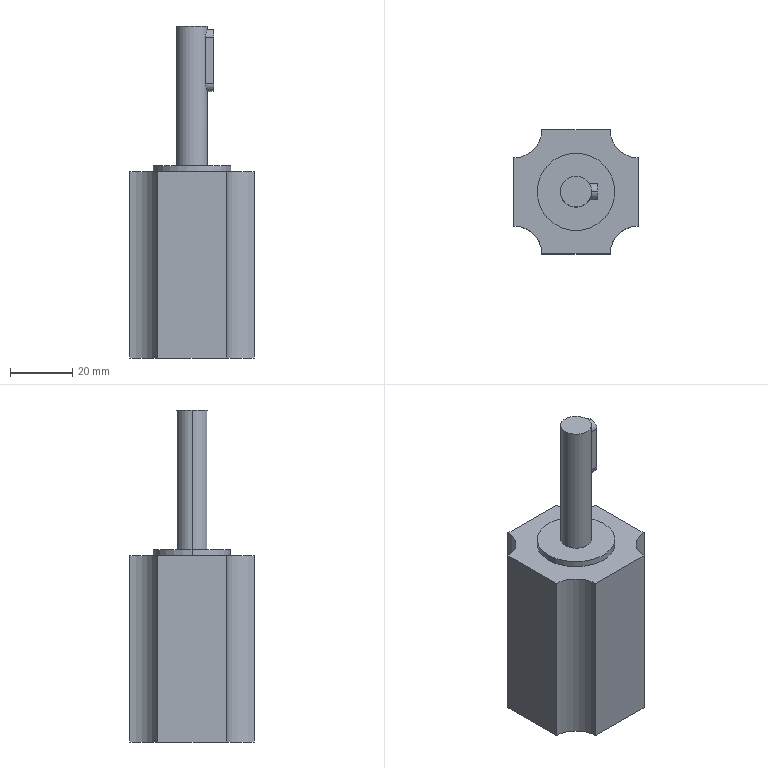Component | SolidWorks | FormingWheelMotor-1 | 1 solid | 22 faces | box 40 x 40 x 107 mm | volume 85457 mm3 | cylinder 11 | plane 11 | commonest cylinder face diameters 18 x4 5 x3 25 x2 10 x2
build123d program:
from build123d import *

# Parameters (mm, degrees)
SKETCH1_R           = 5
BOSS_EXTRUDE1_DEPTH = 45
SKETCH4_R           = 12.5
BOSS_EXTRUDE2_DEPTH = 2
SKETCH5_W           = 40
SKETCH5_H           = 40
BOSS_EXTRUDE3_DEPTH = 60
SKETCH6_R           = 9
CUT_EXTRUDE2_DEPTH  = 111.675
BOSS_EXTRUDE4_DEPTH = 7


with BuildPart() as part:
    # Sketch1 → Boss-Extrude1 (new body)
    with BuildSketch(Plane(origin=(0, 0, 0), x_dir=(0, 0, -1), z_dir=(1, 0, 0))):
        with Locations(Location((0, 0, 0), (0, 0, 180))):
            Circle(SKETCH1_R)
    extrude(amount=BOSS_EXTRUDE1_DEPTH)

    # Sketch4 → Boss-Extrude2 (add)
    with BuildSketch(Plane(origin=(45, 0, 0), x_dir=(0, 0, -1), z_dir=(1, 0, 0))):
        Circle(SKETCH4_R)
    extrude(amount=BOSS_EXTRUDE2_DEPTH)

    # Sketch5 → Boss-Extrude3 (add)
    with BuildSketch(Plane(origin=(47, 0, 0), x_dir=(0, 0, -1), z_dir=(1, 0, 0))):
        Rectangle(SKETCH5_W, SKETCH5_H)
    extrude(amount=BOSS_EXTRUDE3_DEPTH)

    # Sketch6 → Cut-Extrude2 (cut, through all)
    with BuildSketch(Plane(origin=(107, 0, 0), x_dir=(0, 0, -1), z_dir=(1, 0, 0))):
        with Locations((-20, 20)):
            Circle(SKETCH6_R)
        with Locations((20, 20)):
            Circle(SKETCH6_R)
        with Locations((20, -20)):
            Circle(SKETCH6_R)
        with Locations((-20, -20)):
            Circle(SKETCH6_R)
    extrude(amount=-CUT_EXTRUDE2_DEPTH, mode=Mode.SUBTRACT)

    # Sketch3 → Boss-Extrude4 (add)
    with BuildSketch(Plane.XY):
        with BuildLine():
            Line((3.623, 2.5), (18.623, 2.5))
            ThreePointArc((18.623, 2.5), (21.123, 0), (18.623, -2.5))
            Line((18.623, -2.5), (3.623, -2.5))
            ThreePointArc((3.623, -2.5), (1.123, 0), (3.623, 2.5))
        make_face()
    extrude(amount=BOSS_EXTRUDE4_DEPTH)


solid = part.part

# Placed as in the assembly
solid = solid.moved(Location((246.241, -267.715, 1455.724), (0, 90, 0)))
STEP:
#1=CARTESIAN_POINT('',(9.97,-10.54,57.268));
#2=VERTEX_POINT('',#1);
#3=CARTESIAN_POINT('',(9.97,-10.638,57.169));
#4=VERTEX_POINT('',#3);
#5=CARTESIAN_POINT('',(9.97,-10.54,57.169));
#6=DIRECTION('',(1.,0.,-0.));
#7=DIRECTION('',(0.,0.,-1.));
#8=AXIS2_PLACEMENT_3D('',#5,#6,#7);
#9=CIRCLE('',#8,0.09843);
#10=EDGE_CURVE('',#2,#4,#9,.T.);
#11=ORIENTED_EDGE('',*,*,#10,.F.);
#12=CARTESIAN_POINT('',(9.891,-10.54,57.268));
#13=VERTEX_POINT('',#12);
#14=CARTESIAN_POINT('',(9.97,-10.54,57.268));
#15=DIRECTION('',(-1.,-0.,0.));
#16=VECTOR('',#15,39.37);
#17=LINE('',#14,#16);
#18=EDGE_CURVE('',#2,#13,#17,.T.);
#19=ORIENTED_EDGE('',*,*,#18,.T.);
#20=CARTESIAN_POINT('',(9.865,-10.638,57.169));
#21=VERTEX_POINT('',#20);
#22=CARTESIAN_POINT('',(9.891,-10.54,57.268));
#23=CARTESIAN_POINT('',(9.891,-10.546,57.268));
#24=CARTESIAN_POINT('',(9.891,-10.553,57.267));
#25=CARTESIAN_POINT('',(9.89,-10.566,57.265));
#26=CARTESIAN_POINT('',(9.889,-10.572,57.263));
#27=CARTESIAN_POINT('',(9.886,-10.584,57.258));
#28=CARTESIAN_POINT('',(9.885,-10.59,57.255));
#29=CARTESIAN_POINT('',(9.882,-10.6,57.247));
#30=CARTESIAN_POINT('',(9.88,-10.605,57.243));
#31=CARTESIAN_POINT('',(9.877,-10.614,57.234));
#32=CARTESIAN_POINT('',(9.875,-10.618,57.229));
#33=CARTESIAN_POINT('',(9.872,-10.625,57.219));
#34=CARTESIAN_POINT('',(9.87,-10.628,57.213));
#35=CARTESIAN_POINT('',(9.868,-10.633,57.201));
#36=CARTESIAN_POINT('',(9.867,-10.635,57.195));
#37=CARTESIAN_POINT('',(9.865,-10.638,57.182));
#38=CARTESIAN_POINT('',(9.865,-10.638,57.176));
#39=CARTESIAN_POINT('',(9.865,-10.638,57.169));
#40=B_SPLINE_CURVE_WITH_KNOTS('',3,(#22,#23,#24,#25,#26,#27,#28,#29,#30,#31,#32,#33,#34,#35,#36,#37,#38,#39),.UNSPECIFIED.,.F.,.F.,(4,2,2,2,2,2,2,2,4),(0.007952,0.008449,0.008945,0.009442,0.009938,0.01043,0.01093,0.01143,0.01192),.UNSPECIFIED.);
#41=EDGE_CURVE('',#13,#21,#40,.T.);
#42=ORIENTED_EDGE('',*,*,#41,.T.);
#43=CARTESIAN_POINT('',(9.97,-10.638,57.169));
#44=DIRECTION('',(-1.,-0.,0.));
#45=VECTOR('',#44,39.37);
#46=LINE('',#43,#45);
#47=EDGE_CURVE('',#4,#21,#46,.T.);
#48=ORIENTED_EDGE('',*,*,#47,.F.);
#49=EDGE_LOOP('',(#11,#19,#42,#48));
#50=FACE_OUTER_BOUND('',#49,.T.);
#51=CARTESIAN_POINT('',(9.97,-10.54,57.169));
#52=DIRECTION('',(-1.,-0.,0.));
#53=DIRECTION('',(0.,0.,1.));
#54=AXIS2_PLACEMENT_3D('',#51,#52,#53);
#55=CYLINDRICAL_SURFACE('',#54,0.09843);
#56=ADVANCED_FACE('',(#50),#55,.T.);
#57=CARTESIAN_POINT('',(9.202,-10.54,55.462));
#58=VERTEX_POINT('',#57);
#59=CARTESIAN_POINT('',(10.187,-10.54,55.462));
#60=VERTEX_POINT('',#59);
#61=CARTESIAN_POINT('',(9.695,-10.54,55.462));
#62=DIRECTION('',(-0.,0.,-1.));
#63=DIRECTION('',(-1.,0.,0.));
#64=AXIS2_PLACEMENT_3D('',#61,#62,#63);
#65=CIRCLE('',#64,0.4921);
#66=EDGE_CURVE('',#58,#60,#65,.T.);
#67=ORIENTED_EDGE('',*,*,#66,.F.);
#68=CARTESIAN_POINT('',(9.202,-10.54,55.54));
#69=VERTEX_POINT('',#68);
#70=CARTESIAN_POINT('',(9.202,-10.54,55.462));
#71=DIRECTION('',(0.,-0.,1.));
#72=VECTOR('',#71,39.37);
#73=LINE('',#70,#72);
#74=EDGE_CURVE('',#58,#69,#73,.T.);
#75=ORIENTED_EDGE('',*,*,#74,.T.);
#76=CARTESIAN_POINT('',(10.187,-10.54,55.54));
#77=VERTEX_POINT('',#76);
#78=CARTESIAN_POINT('',(9.695,-10.54,55.54));
#79=DIRECTION('',(-0.,0.,-1.));
#80=DIRECTION('',(-1.,0.,0.));
#81=AXIS2_PLACEMENT_3D('',#78,#79,#80);
#82=CIRCLE('',#81,0.4921);
#83=EDGE_CURVE('',#69,#77,#82,.T.);
#84=ORIENTED_EDGE('',*,*,#83,.T.);
#85=CARTESIAN_POINT('',(10.187,-10.54,55.462));
#86=DIRECTION('',(0.,-0.,1.));
#87=VECTOR('',#86,39.37);
#88=LINE('',#85,#87);
#89=EDGE_CURVE('',#60,#77,#88,.T.);
#90=ORIENTED_EDGE('',*,*,#89,.F.);
#91=EDGE_LOOP('',(#67,#75,#84,#90));
#92=FACE_OUTER_BOUND('',#91,.T.);
#93=CARTESIAN_POINT('',(9.695,-10.54,55.462));
#94=DIRECTION('',(0.,-0.,1.));
#95=DIRECTION('',(1.,0.,0.));
#96=AXIS2_PLACEMENT_3D('',#93,#94,#95);
#97=CYLINDRICAL_SURFACE('',#96,0.4921);
#98=ADVANCED_FACE('',(#92),#97,.T.);
#99=CARTESIAN_POINT('',(9.498,-10.54,55.54));
#100=VERTEX_POINT('',#99);
#101=CARTESIAN_POINT('',(9.891,-10.54,55.54));
#102=VERTEX_POINT('',#101);
#103=CARTESIAN_POINT('',(9.695,-10.54,55.54));
#104=DIRECTION('',(-0.,0.,-1.));
#105=DIRECTION('',(-1.,0.,0.));
#106=AXIS2_PLACEMENT_3D('',#103,#104,#105);
#107=CIRCLE('',#106,0.1969);
#108=EDGE_CURVE('',#100,#102,#107,.T.);
#109=ORIENTED_EDGE('',*,*,#108,.F.);
#110=CARTESIAN_POINT('',(9.498,-10.54,57.312));
#111=VERTEX_POINT('',#110);
#112=CARTESIAN_POINT('',(9.498,-10.54,55.54));
#113=DIRECTION('',(0.,-0.,1.));
#114=VECTOR('',#113,39.37);
#115=LINE('',#112,#114);
#116=EDGE_CURVE('',#100,#111,#115,.T.);
#117=ORIENTED_EDGE('',*,*,#116,.T.);
#118=CARTESIAN_POINT('',(9.891,-10.54,57.312));
#119=VERTEX_POINT('',#118);
#120=CARTESIAN_POINT('',(9.695,-10.54,57.312));
#121=DIRECTION('',(-0.,0.,-1.));
#122=DIRECTION('',(-1.,0.,0.));
#123=AXIS2_PLACEMENT_3D('',#120,#121,#122);
#124=CIRCLE('',#123,0.1969);
#125=EDGE_CURVE('',#111,#119,#124,.T.);
#126=ORIENTED_EDGE('',*,*,#125,.T.);
#127=CARTESIAN_POINT('',(9.891,-10.54,55.54));
#128=DIRECTION('',(0.,-0.,1.));
#129=VECTOR('',#128,39.37);
#130=LINE('',#127,#129);
#131=EDGE_CURVE('',#13,#119,#130,.T.);
#132=ORIENTED_EDGE('',*,*,#131,.F.);
#133=CARTESIAN_POINT('',(9.865,-10.442,57.169));
#134=VERTEX_POINT('',#133);
#135=CARTESIAN_POINT('',(9.865,-10.442,57.169));
#136=CARTESIAN_POINT('',(9.865,-10.442,57.176));
#137=CARTESIAN_POINT('',(9.865,-10.442,57.183));
#138=CARTESIAN_POINT('',(9.867,-10.445,57.195));
#139=CARTESIAN_POINT('',(9.868,-10.447,57.202));
#140=CARTESIAN_POINT('',(9.871,-10.452,57.213));
#141=CARTESIAN_POINT('',(9.872,-10.455,57.219));
#142=CARTESIAN_POINT('',(9.875,-10.462,57.23));
#143=CARTESIAN_POINT('',(9.877,-10.466,57.235));
#144=CARTESIAN_POINT('',(9.882,-10.479,57.248));
#145=CARTESIAN_POINT('',(9.885,-10.49,57.255));
#146=CARTESIAN_POINT('',(9.889,-10.508,57.263));
#147=CARTESIAN_POINT('',(9.89,-10.514,57.265));
#148=CARTESIAN_POINT('',(9.891,-10.527,57.267));
#149=CARTESIAN_POINT('',(9.891,-10.533,57.268));
#150=CARTESIAN_POINT('',(9.891,-10.54,57.268));
#151=B_SPLINE_CURVE_WITH_KNOTS('',3,(#135,#136,#137,#138,#139,#140,#141,#142,#143,#144,#145,#146,#147,#148,#149,#150),.UNSPECIFIED.,.F.,.F.,(4,2,2,2,2,2,2,4),(0.003979,0.004475,0.004972,0.005469,0.005966,0.006959,0.007456,0.007952),.UNSPECIFIED.);
#152=EDGE_CURVE('',#134,#13,#151,.T.);
#153=ORIENTED_EDGE('',*,*,#152,.F.);
#154=CARTESIAN_POINT('',(9.865,-10.442,56.579));
#155=VERTEX_POINT('',#154);
#156=CARTESIAN_POINT('',(9.865,-10.442,55.54));
#157=DIRECTION('',(0.,-0.,1.));
#158=VECTOR('',#157,39.37);
#159=LINE('',#156,#158);
#160=EDGE_CURVE('',#155,#134,#159,.T.);
#161=ORIENTED_EDGE('',*,*,#160,.F.);
#162=CARTESIAN_POINT('',(9.891,-10.54,56.48));
#163=VERTEX_POINT('',#162);
#164=CARTESIAN_POINT('',(9.891,-10.54,56.48));
#165=CARTESIAN_POINT('',(9.891,-10.533,56.48));
#166=CARTESIAN_POINT('',(9.891,-10.527,56.481));
#167=CARTESIAN_POINT('',(9.89,-10.514,56.484));
#168=CARTESIAN_POINT('',(9.889,-10.508,56.486));
#169=CARTESIAN_POINT('',(9.885,-10.49,56.493));
#170=CARTESIAN_POINT('',(9.882,-10.479,56.5));
#171=CARTESIAN_POINT('',(9.877,-10.466,56.514));
#172=CARTESIAN_POINT('',(9.875,-10.462,56.519));
#173=CARTESIAN_POINT('',(9.872,-10.455,56.529));
#174=CARTESIAN_POINT('',(9.87,-10.452,56.535));
#175=CARTESIAN_POINT('',(9.868,-10.447,56.547));
#176=CARTESIAN_POINT('',(9.867,-10.445,56.553));
#177=CARTESIAN_POINT('',(9.865,-10.442,56.566));
#178=CARTESIAN_POINT('',(9.865,-10.442,56.572));
#179=CARTESIAN_POINT('',(9.865,-10.442,56.579));
#180=B_SPLINE_CURVE_WITH_KNOTS('',3,(#164,#165,#166,#167,#168,#169,#170,#171,#172,#173,#174,#175,#176,#177,#178,#179),.UNSPECIFIED.,.F.,.F.,(4,2,2,2,2,2,2,4),(0.,0.0004973,0.0009947,0.001989,0.002487,0.002984,0.003481,0.003979),.UNSPECIFIED.);
#181=EDGE_CURVE('',#163,#155,#180,.T.);
#182=ORIENTED_EDGE('',*,*,#181,.F.);
#183=CARTESIAN_POINT('',(9.891,-10.54,55.54));
#184=DIRECTION('',(0.,-0.,1.));
#185=VECTOR('',#184,39.37);
#186=LINE('',#183,#185);
#187=EDGE_CURVE('',#102,#163,#186,.T.);
#188=ORIENTED_EDGE('',*,*,#187,.F.);
#189=EDGE_LOOP('',(#109,#117,#126,#132,#153,#161,#182,#188));
#190=FACE_OUTER_BOUND('',#189,.T.);
#191=CARTESIAN_POINT('',(9.695,-10.54,55.54));
#192=DIRECTION('',(0.,-0.,1.));
#193=DIRECTION('',(1.,0.,0.));
#194=AXIS2_PLACEMENT_3D('',#191,#192,#193);
#195=CYLINDRICAL_SURFACE('',#194,0.1969);
#196=ADVANCED_FACE('',(#190),#195,.T.);
#197=ORIENTED_EDGE('',*,*,#116,.F.);
#198=CARTESIAN_POINT('',(9.695,-10.54,55.54));
#199=DIRECTION('',(-0.,0.,-1.));
#200=DIRECTION('',(-1.,0.,0.));
#201=AXIS2_PLACEMENT_3D('',#198,#199,#200);
#202=CIRCLE('',#201,0.1969);
#203=EDGE_CURVE('',#102,#100,#202,.T.);
#204=ORIENTED_EDGE('',*,*,#203,.F.);
#205=ORIENTED_EDGE('',*,*,#187,.T.);
#206=CARTESIAN_POINT('',(9.865,-10.638,56.579));
#207=VERTEX_POINT('',#206);
#208=CARTESIAN_POINT('',(9.865,-10.638,56.579));
#209=CARTESIAN_POINT('',(9.865,-10.638,56.572));
#210=CARTESIAN_POINT('',(9.865,-10.638,56.566));
#211=CARTESIAN_POINT('',(9.867,-10.635,56.553));
#212=CARTESIAN_POINT('',(9.868,-10.633,56.547));
#213=CARTESIAN_POINT('',(9.872,-10.626,56.529));
#214=CARTESIAN_POINT('',(9.875,-10.619,56.518));
#215=CARTESIAN_POINT('',(9.88,-10.605,56.505));
#216=CARTESIAN_POINT('',(9.882,-10.6,56.501));
#217=CARTESIAN_POINT('',(9.885,-10.59,56.494));
#218=CARTESIAN_POINT('',(9.886,-10.584,56.491));
#219=CARTESIAN_POINT('',(9.889,-10.572,56.486));
#220=CARTESIAN_POINT('',(9.89,-10.566,56.484));
#221=CARTESIAN_POINT('',(9.891,-10.553,56.481));
#222=CARTESIAN_POINT('',(9.891,-10.547,56.48));
#223=CARTESIAN_POINT('',(9.891,-10.54,56.48));
#224=B_SPLINE_CURVE_WITH_KNOTS('',3,(#208,#209,#210,#211,#212,#213,#214,#215,#216,#217,#218,#219,#220,#221,#222,#223),.UNSPECIFIED.,.F.,.F.,(4,2,2,2,2,2,2,4),(0.01192,0.01242,0.01292,0.01391,0.0144,0.0149,0.0154,0.01589),.UNSPECIFIED.);
#225=EDGE_CURVE('',#207,#163,#224,.T.);
#226=ORIENTED_EDGE('',*,*,#225,.F.);
#227=CARTESIAN_POINT('',(9.865,-10.638,55.54));
#228=DIRECTION('',(-0.,0.,-1.));
#229=VECTOR('',#228,39.37);
#230=LINE('',#227,#229);
#231=EDGE_CURVE('',#21,#207,#230,.T.);
#232=ORIENTED_EDGE('',*,*,#231,.F.);
#233=ORIENTED_EDGE('',*,*,#41,.F.);
#234=ORIENTED_EDGE('',*,*,#131,.T.);
#235=CARTESIAN_POINT('',(9.695,-10.54,57.312));
#236=DIRECTION('',(-0.,0.,-1.));
#237=DIRECTION('',(-1.,0.,0.));
#238=AXIS2_PLACEMENT_3D('',#235,#236,#237);
#239=CIRCLE('',#238,0.1969);
#240=EDGE_CURVE('',#119,#111,#239,.T.);
#241=ORIENTED_EDGE('',*,*,#240,.T.);
#242=EDGE_LOOP('',(#197,#204,#205,#226,#232,#233,#234,#241));
#243=FACE_OUTER_BOUND('',#242,.T.);
#244=CARTESIAN_POINT('',(9.695,-10.54,55.54));
#245=DIRECTION('',(0.,-0.,1.));
#246=DIRECTION('',(1.,0.,0.));
#247=AXIS2_PLACEMENT_3D('',#244,#245,#246);
#248=CYLINDRICAL_SURFACE('',#247,0.1969);
#249=ADVANCED_FACE('',(#243),#248,.T.);
#250=ORIENTED_EDGE('',*,*,#240,.F.);
#251=ORIENTED_EDGE('',*,*,#125,.F.);
#252=EDGE_LOOP('',(#250,#251));
#253=FACE_OUTER_BOUND('',#252,.T.);
#254=CARTESIAN_POINT('',(9.695,-10.54,57.312));
#255=DIRECTION('',(-0.,0.,-1.));
#256=DIRECTION('',(-1.,-0.,0.));
#257=AXIS2_PLACEMENT_3D('',#254,#255,#256);
#258=PLANE('',#257);
#259=ADVANCED_FACE('',(#253),#258,.F.);
#260=CARTESIAN_POINT('',(9.695,-10.54,55.54));
#261=DIRECTION('',(-0.,0.,-1.));
#262=DIRECTION('',(-1.,0.,0.));
#263=AXIS2_PLACEMENT_3D('',#260,#261,#262);
#264=CIRCLE('',#263,0.4921);
#265=EDGE_CURVE('',#77,#69,#264,.T.);
#266=ORIENTED_EDGE('',*,*,#265,.F.);
#267=ORIENTED_EDGE('',*,*,#83,.F.);
#268=EDGE_LOOP('',(#266,#267));
#269=FACE_OUTER_BOUND('',#268,.T.);
#270=ORIENTED_EDGE('',*,*,#203,.T.);
#271=ORIENTED_EDGE('',*,*,#108,.T.);
#272=EDGE_LOOP('',(#270,#271));
#273=FACE_BOUND('',#272,.T.);
#274=CARTESIAN_POINT('',(9.695,-10.54,55.54));
#275=DIRECTION('',(-0.,0.,-1.));
#276=DIRECTION('',(-1.,-0.,0.));
#277=AXIS2_PLACEMENT_3D('',#274,#275,#276);
#278=PLANE('',#277);
#279=ADVANCED_FACE('',(#269,#273),#278,.F.);
#280=ORIENTED_EDGE('',*,*,#74,.F.);
#281=CARTESIAN_POINT('',(9.695,-10.54,55.462));
#282=DIRECTION('',(-0.,0.,-1.));
#283=DIRECTION('',(-1.,0.,0.));
#284=AXIS2_PLACEMENT_3D('',#281,#282,#283);
#285=CIRCLE('',#284,0.4921);
#286=EDGE_CURVE('',#60,#58,#285,.T.);
#287=ORIENTED_EDGE('',*,*,#286,.F.);
#288=ORIENTED_EDGE('',*,*,#89,.T.);
#289=ORIENTED_EDGE('',*,*,#265,.T.);
#290=EDGE_LOOP('',(#280,#287,#288,#289));
#291=FACE_OUTER_BOUND('',#290,.T.);
#292=CARTESIAN_POINT('',(9.695,-10.54,55.462));
#293=DIRECTION('',(0.,-0.,1.));
#294=DIRECTION('',(1.,0.,0.));
#295=AXIS2_PLACEMENT_3D('',#292,#293,#294);
#296=CYLINDRICAL_SURFACE('',#295,0.4921);
#297=ADVANCED_FACE('',(#291),#296,.T.);
#298=CARTESIAN_POINT('',(10.128,-11.327,55.462));
#299=VERTEX_POINT('',#298);
#300=CARTESIAN_POINT('',(9.261,-11.327,55.462));
#301=VERTEX_POINT('',#300);
#302=CARTESIAN_POINT('',(8.907,-11.327,55.462));
#303=DIRECTION('',(-1.,0.,0.));
#304=VECTOR('',#303,39.37);
#305=LINE('',#302,#304);
#306=EDGE_CURVE('',#299,#301,#305,.T.);
#307=ORIENTED_EDGE('',*,*,#306,.F.);
#308=CARTESIAN_POINT('',(10.482,-10.973,55.462));
#309=VERTEX_POINT('',#308);
#310=CARTESIAN_POINT('',(10.482,-11.327,55.462));
#311=DIRECTION('',(-0.,0.,-1.));
#312=DIRECTION('',(-1.,0.,0.));
#313=AXIS2_PLACEMENT_3D('',#310,#311,#312);
#314=CIRCLE('',#313,0.3543);
#315=EDGE_CURVE('',#299,#309,#314,.T.);
#316=ORIENTED_EDGE('',*,*,#315,.T.);
#317=CARTESIAN_POINT('',(10.482,-10.107,55.462));
#318=VERTEX_POINT('',#317);
#319=CARTESIAN_POINT('',(10.482,-11.327,55.462));
#320=DIRECTION('',(0.,-1.,-0.));
#321=VECTOR('',#320,39.37);
#322=LINE('',#319,#321);
#323=EDGE_CURVE('',#318,#309,#322,.T.);
#324=ORIENTED_EDGE('',*,*,#323,.F.);
#325=CARTESIAN_POINT('',(10.128,-9.753,55.462));
#326=VERTEX_POINT('',#325);
#327=CARTESIAN_POINT('',(10.482,-9.753,55.462));
#328=DIRECTION('',(-0.,0.,-1.));
#329=DIRECTION('',(-1.,0.,0.));
#330=AXIS2_PLACEMENT_3D('',#327,#328,#329);
#331=CIRCLE('',#330,0.3543);
#332=EDGE_CURVE('',#318,#326,#331,.T.);
#333=ORIENTED_EDGE('',*,*,#332,.T.);
#334=CARTESIAN_POINT('',(9.261,-9.753,55.462));
#335=VERTEX_POINT('',#334);
#336=CARTESIAN_POINT('',(8.907,-9.753,55.462));
#337=DIRECTION('',(1.,-0.,-0.));
#338=VECTOR('',#337,39.37);
#339=LINE('',#336,#338);
#340=EDGE_CURVE('',#335,#326,#339,.T.);
#341=ORIENTED_EDGE('',*,*,#340,.F.);
#342=CARTESIAN_POINT('',(8.907,-10.107,55.462));
#343=VERTEX_POINT('',#342);
#344=CARTESIAN_POINT('',(8.907,-9.753,55.462));
#345=DIRECTION('',(-0.,0.,-1.));
#346=DIRECTION('',(-1.,0.,0.));
#347=AXIS2_PLACEMENT_3D('',#344,#345,#346);
#348=CIRCLE('',#347,0.3543);
#349=EDGE_CURVE('',#335,#343,#348,.T.);
#350=ORIENTED_EDGE('',*,*,#349,.T.);
#351=CARTESIAN_POINT('',(8.907,-10.973,55.462));
#352=VERTEX_POINT('',#351);
#353=CARTESIAN_POINT('',(8.907,-11.327,55.462));
#354=DIRECTION('',(-0.,1.,0.));
#355=VECTOR('',#354,39.37);
#356=LINE('',#353,#355);
#357=EDGE_CURVE('',#352,#343,#356,.T.);
#358=ORIENTED_EDGE('',*,*,#357,.F.);
#359=CARTESIAN_POINT('',(8.907,-11.327,55.462));
#360=DIRECTION('',(-0.,0.,-1.));
#361=DIRECTION('',(-1.,0.,0.));
#362=AXIS2_PLACEMENT_3D('',#359,#360,#361);
#363=CIRCLE('',#362,0.3543);
#364=EDGE_CURVE('',#352,#301,#363,.T.);
#365=ORIENTED_EDGE('',*,*,#364,.T.);
#366=EDGE_LOOP('',(#307,#316,#324,#333,#341,#350,#358,#365));
#367=FACE_OUTER_BOUND('',#366,.T.);
#368=ORIENTED_EDGE('',*,*,#286,.T.);
#369=ORIENTED_EDGE('',*,*,#66,.T.);
#370=EDGE_LOOP('',(#368,#369));
#371=FACE_BOUND('',#370,.T.);
#372=CARTESIAN_POINT('',(9.695,-10.54,55.462));
#373=DIRECTION('',(-0.,0.,-1.));
#374=DIRECTION('',(-1.,-0.,0.));
#375=AXIS2_PLACEMENT_3D('',#372,#373,#374);
#376=PLANE('',#375);
#377=ADVANCED_FACE('',(#367,#371),#376,.F.);
#378=ORIENTED_EDGE('',*,*,#323,.T.);
#379=CARTESIAN_POINT('',(10.482,-10.973,53.099));
#380=VERTEX_POINT('',#379);
#381=CARTESIAN_POINT('',(10.482,-10.973,57.312));
#382=DIRECTION('',(-0.,0.,-1.));
#383=VECTOR('',#382,39.37);
#384=LINE('',#381,#383);
#385=EDGE_CURVE('',#309,#380,#384,.T.);
#386=ORIENTED_EDGE('',*,*,#385,.T.);
#387=CARTESIAN_POINT('',(10.482,-10.107,53.099));
#388=VERTEX_POINT('',#387);
#389=CARTESIAN_POINT('',(10.482,-11.327,53.099));
#390=DIRECTION('',(0.,-1.,-0.));
#391=VECTOR('',#390,39.37);
#392=LINE('',#389,#391);
#393=EDGE_CURVE('',#388,#380,#392,.T.);
#394=ORIENTED_EDGE('',*,*,#393,.F.);
#395=CARTESIAN_POINT('',(10.482,-10.107,57.312));
#396=DIRECTION('',(0.,-0.,1.));
#397=VECTOR('',#396,39.37);
#398=LINE('',#395,#397);
#399=EDGE_CURVE('',#388,#318,#398,.T.);
#400=ORIENTED_EDGE('',*,*,#399,.T.);
#401=EDGE_LOOP('',(#378,#386,#394,#400));
#402=FACE_OUTER_BOUND('',#401,.T.);
#403=CARTESIAN_POINT('',(10.482,-11.327,53.099));
#404=DIRECTION('',(-1.,-0.,0.));
#405=DIRECTION('',(0.,-0.,1.));
#406=AXIS2_PLACEMENT_3D('',#403,#404,#405);
#407=PLANE('',#406);
#408=ADVANCED_FACE('',(#402),#407,.F.);
#409=CARTESIAN_POINT('',(10.128,-11.327,53.099));
#410=VERTEX_POINT('',#409);
#411=CARTESIAN_POINT('',(9.261,-11.327,53.099));
#412=VERTEX_POINT('',#411);
#413=CARTESIAN_POINT('',(8.907,-11.327,53.099));
#414=DIRECTION('',(-1.,0.,0.));
#415=VECTOR('',#414,39.37);
#416=LINE('',#413,#415);
#417=EDGE_CURVE('',#410,#412,#416,.T.);
#418=ORIENTED_EDGE('',*,*,#417,.F.);
#419=CARTESIAN_POINT('',(10.128,-11.327,57.312));
#420=DIRECTION('',(0.,-0.,1.));
#421=VECTOR('',#420,39.37);
#422=LINE('',#419,#421);
#423=EDGE_CURVE('',#410,#299,#422,.T.);
#424=ORIENTED_EDGE('',*,*,#423,.T.);
#425=ORIENTED_EDGE('',*,*,#306,.T.);
#426=CARTESIAN_POINT('',(9.261,-11.327,57.312));
#427=DIRECTION('',(-0.,0.,-1.));
#428=VECTOR('',#427,39.37);
#429=LINE('',#426,#428);
#430=EDGE_CURVE('',#301,#412,#429,.T.);
#431=ORIENTED_EDGE('',*,*,#430,.T.);
#432=EDGE_LOOP('',(#418,#424,#425,#431));
#433=FACE_OUTER_BOUND('',#432,.T.);
#434=CARTESIAN_POINT('',(8.907,-11.327,53.099));
#435=DIRECTION('',(0.,1.,0.));
#436=DIRECTION('',(1.,-0.,-0.));
#437=AXIS2_PLACEMENT_3D('',#434,#435,#436);
#438=PLANE('',#437);
#439=ADVANCED_FACE('',(#433),#438,.F.);
#440=CARTESIAN_POINT('',(8.907,-10.973,53.099));
#441=VERTEX_POINT('',#440);
#442=CARTESIAN_POINT('',(8.907,-10.107,53.099));
#443=VERTEX_POINT('',#442);
#444=CARTESIAN_POINT('',(8.907,-11.327,53.099));
#445=DIRECTION('',(-0.,1.,0.));
#446=VECTOR('',#445,39.37);
#447=LINE('',#444,#446);
#448=EDGE_CURVE('',#441,#443,#447,.T.);
#449=ORIENTED_EDGE('',*,*,#448,.F.);
#450=CARTESIAN_POINT('',(8.907,-10.973,57.312));
#451=DIRECTION('',(0.,-0.,1.));
#452=VECTOR('',#451,39.37);
#453=LINE('',#450,#452);
#454=EDGE_CURVE('',#441,#352,#453,.T.);
#455=ORIENTED_EDGE('',*,*,#454,.T.);
#456=ORIENTED_EDGE('',*,*,#357,.T.);
#457=CARTESIAN_POINT('',(8.907,-10.107,57.312));
#458=DIRECTION('',(-0.,0.,-1.));
#459=VECTOR('',#458,39.37);
#460=LINE('',#457,#459);
#461=EDGE_CURVE('',#343,#443,#460,.T.);
#462=ORIENTED_EDGE('',*,*,#461,.T.);
#463=EDGE_LOOP('',(#449,#455,#456,#462));
#464=FACE_OUTER_BOUND('',#463,.T.);
#465=CARTESIAN_POINT('',(8.907,-11.327,53.099));
#466=DIRECTION('',(1.,0.,-0.));
#467=DIRECTION('',(-0.,0.,-1.));
#468=AXIS2_PLACEMENT_3D('',#465,#466,#467);
#469=PLANE('',#468);
#470=ADVANCED_FACE('',(#464),#469,.F.);
#471=CARTESIAN_POINT('',(9.261,-9.753,53.099));
#472=VERTEX_POINT('',#471);
#473=CARTESIAN_POINT('',(10.128,-9.753,53.099));
#474=VERTEX_POINT('',#473);
#475=CARTESIAN_POINT('',(8.907,-9.753,53.099));
#476=DIRECTION('',(1.,-0.,-0.));
#477=VECTOR('',#476,39.37);
#478=LINE('',#475,#477);
#479=EDGE_CURVE('',#472,#474,#478,.T.);
#480=ORIENTED_EDGE('',*,*,#479,.F.);
#481=CARTESIAN_POINT('',(9.261,-9.753,57.312));
#482=DIRECTION('',(0.,-0.,1.));
#483=VECTOR('',#482,39.37);
#484=LINE('',#481,#483);
#485=EDGE_CURVE('',#472,#335,#484,.T.);
#486=ORIENTED_EDGE('',*,*,#485,.T.);
#487=ORIENTED_EDGE('',*,*,#340,.T.);
#488=CARTESIAN_POINT('',(10.128,-9.753,57.312));
#489=DIRECTION('',(-0.,0.,-1.));
#490=VECTOR('',#489,39.37);
#491=LINE('',#488,#490);
#492=EDGE_CURVE('',#326,#474,#491,.T.);
#493=ORIENTED_EDGE('',*,*,#492,.T.);
#494=EDGE_LOOP('',(#480,#486,#487,#493));
#495=FACE_OUTER_BOUND('',#494,.T.);
#496=CARTESIAN_POINT('',(8.907,-9.753,53.099));
#497=DIRECTION('',(-0.,-1.,-0.));
#498=DIRECTION('',(-1.,0.,0.));
#499=AXIS2_PLACEMENT_3D('',#496,#497,#498);
#500=PLANE('',#499);
#501=ADVANCED_FACE('',(#495),#500,.F.);
#502=CARTESIAN_POINT('',(10.482,-11.327,53.099));
#503=DIRECTION('',(-0.,0.,-1.));
#504=DIRECTION('',(-1.,0.,0.));
#505=AXIS2_PLACEMENT_3D('',#502,#503,#504);
#506=CIRCLE('',#505,0.3543);
#507=EDGE_CURVE('',#410,#380,#506,.T.);
#508=ORIENTED_EDGE('',*,*,#507,.F.);
#509=ORIENTED_EDGE('',*,*,#417,.T.);
#510=CARTESIAN_POINT('',(8.907,-11.327,53.099));
#511=DIRECTION('',(-0.,0.,-1.));
#512=DIRECTION('',(-1.,0.,0.));
#513=AXIS2_PLACEMENT_3D('',#510,#511,#512);
#514=CIRCLE('',#513,0.3543);
#515=EDGE_CURVE('',#441,#412,#514,.T.);
#516=ORIENTED_EDGE('',*,*,#515,.F.);
#517=ORIENTED_EDGE('',*,*,#448,.T.);
#518=CARTESIAN_POINT('',(8.907,-9.753,53.099));
#519=DIRECTION('',(-0.,0.,-1.));
#520=DIRECTION('',(-1.,0.,0.));
#521=AXIS2_PLACEMENT_3D('',#518,#519,#520);
#522=CIRCLE('',#521,0.3543);
#523=EDGE_CURVE('',#472,#443,#522,.T.);
#524=ORIENTED_EDGE('',*,*,#523,.F.);
#525=ORIENTED_EDGE('',*,*,#479,.T.);
#526=CARTESIAN_POINT('',(10.482,-9.753,53.099));
#527=DIRECTION('',(-0.,0.,-1.));
#528=DIRECTION('',(-1.,0.,0.));
#529=AXIS2_PLACEMENT_3D('',#526,#527,#528);
#530=CIRCLE('',#529,0.3543);
#531=EDGE_CURVE('',#388,#474,#530,.T.);
#532=ORIENTED_EDGE('',*,*,#531,.F.);
#533=ORIENTED_EDGE('',*,*,#393,.T.);
#534=EDGE_LOOP('',(#508,#509,#516,#517,#524,#525,#532,#533));
#535=FACE_OUTER_BOUND('',#534,.T.);
#536=CARTESIAN_POINT('',(9.695,-10.54,53.099));
#537=DIRECTION('',(-0.,0.,-1.));
#538=DIRECTION('',(-1.,-0.,0.));
#539=AXIS2_PLACEMENT_3D('',#536,#537,#538);
#540=PLANE('',#539);
#541=ADVANCED_FACE('',(#535),#540,.T.);
#542=ORIENTED_EDGE('',*,*,#531,.T.);
#543=ORIENTED_EDGE('',*,*,#492,.F.);
#544=ORIENTED_EDGE('',*,*,#332,.F.);
#545=ORIENTED_EDGE('',*,*,#399,.F.);
#546=EDGE_LOOP('',(#542,#543,#544,#545));
#547=FACE_OUTER_BOUND('',#546,.T.);
#548=CARTESIAN_POINT('',(10.482,-9.753,57.312));
#549=DIRECTION('',(-0.,0.,-1.));
#550=DIRECTION('',(-1.,0.,0.));
#551=AXIS2_PLACEMENT_3D('',#548,#549,#550);
#552=CYLINDRICAL_SURFACE('',#551,0.3543);
#553=ADVANCED_FACE('',(#547),#552,.F.);
#554=ORIENTED_EDGE('',*,*,#349,.F.);
#555=ORIENTED_EDGE('',*,*,#485,.F.);
#556=ORIENTED_EDGE('',*,*,#523,.T.);
#557=ORIENTED_EDGE('',*,*,#461,.F.);
#558=EDGE_LOOP('',(#554,#555,#556,#557));
#559=FACE_OUTER_BOUND('',#558,.T.);
#560=CARTESIAN_POINT('',(8.907,-9.753,57.312));
#561=DIRECTION('',(-0.,0.,-1.));
#562=DIRECTION('',(-1.,0.,0.));
#563=AXIS2_PLACEMENT_3D('',#560,#561,#562);
#564=CYLINDRICAL_SURFACE('',#563,0.3543);
#565=ADVANCED_FACE('',(#559),#564,.F.);
#566=ORIENTED_EDGE('',*,*,#364,.F.);
#567=ORIENTED_EDGE('',*,*,#454,.F.);
#568=ORIENTED_EDGE('',*,*,#515,.T.);
#569=ORIENTED_EDGE('',*,*,#430,.F.);
#570=EDGE_LOOP('',(#566,#567,#568,#569));
#571=FACE_OUTER_BOUND('',#570,.T.);
#572=CARTESIAN_POINT('',(8.907,-11.327,57.312));
#573=DIRECTION('',(-0.,0.,-1.));
#574=DIRECTION('',(-1.,0.,0.));
#575=AXIS2_PLACEMENT_3D('',#572,#573,#574);
#576=CYLINDRICAL_SURFACE('',#575,0.3543);
#577=ADVANCED_FACE('',(#571),#576,.F.);
#578=ORIENTED_EDGE('',*,*,#315,.F.);
#579=ORIENTED_EDGE('',*,*,#423,.F.);
#580=ORIENTED_EDGE('',*,*,#507,.T.);
#581=ORIENTED_EDGE('',*,*,#385,.F.);
#582=EDGE_LOOP('',(#578,#579,#580,#581));
#583=FACE_OUTER_BOUND('',#582,.T.);
#584=CARTESIAN_POINT('',(10.482,-11.327,57.312));
#585=DIRECTION('',(-0.,0.,-1.));
#586=DIRECTION('',(-1.,0.,0.));
#587=AXIS2_PLACEMENT_3D('',#584,#585,#586);
#588=CYLINDRICAL_SURFACE('',#587,0.3543);
#589=ADVANCED_FACE('',(#583),#588,.F.);
#590=ORIENTED_EDGE('',*,*,#18,.F.);
#591=CARTESIAN_POINT('',(9.97,-10.442,57.169));
#592=VERTEX_POINT('',#591);
#593=CARTESIAN_POINT('',(9.97,-10.54,57.169));
#594=DIRECTION('',(1.,0.,-0.));
#595=DIRECTION('',(0.,0.,-1.));
#596=AXIS2_PLACEMENT_3D('',#593,#594,#595);
#597=CIRCLE('',#596,0.09843);
#598=EDGE_CURVE('',#592,#2,#597,.T.);
#599=ORIENTED_EDGE('',*,*,#598,.F.);
#600=CARTESIAN_POINT('',(9.97,-10.442,57.169));
#601=DIRECTION('',(-1.,-0.,0.));
#602=VECTOR('',#601,39.37);
#603=LINE('',#600,#602);
#604=EDGE_CURVE('',#592,#134,#603,.T.);
#605=ORIENTED_EDGE('',*,*,#604,.T.);
#606=ORIENTED_EDGE('',*,*,#152,.T.);
#607=EDGE_LOOP('',(#590,#599,#605,#606));
#608=FACE_OUTER_BOUND('',#607,.T.);
#609=CARTESIAN_POINT('',(9.97,-10.54,57.169));
#610=DIRECTION('',(-1.,-0.,0.));
#611=DIRECTION('',(0.,0.,1.));
#612=AXIS2_PLACEMENT_3D('',#609,#610,#611);
#613=CYLINDRICAL_SURFACE('',#612,0.09843);
#614=ADVANCED_FACE('',(#608),#613,.T.);
#615=ORIENTED_EDGE('',*,*,#47,.T.);
#616=ORIENTED_EDGE('',*,*,#231,.T.);
#617=CARTESIAN_POINT('',(9.97,-10.638,56.579));
#618=VERTEX_POINT('',#617);
#619=CARTESIAN_POINT('',(9.97,-10.638,56.579));
#620=DIRECTION('',(-1.,-0.,0.));
#621=VECTOR('',#620,39.37);
#622=LINE('',#619,#621);
#623=EDGE_CURVE('',#618,#207,#622,.T.);
#624=ORIENTED_EDGE('',*,*,#623,.F.);
#625=CARTESIAN_POINT('',(9.97,-10.638,57.169));
#626=DIRECTION('',(-0.,0.,-1.));
#627=VECTOR('',#626,39.37);
#628=LINE('',#625,#627);
#629=EDGE_CURVE('',#4,#618,#628,.T.);
#630=ORIENTED_EDGE('',*,*,#629,.F.);
#631=EDGE_LOOP('',(#615,#616,#624,#630));
#632=FACE_OUTER_BOUND('',#631,.T.);
#633=CARTESIAN_POINT('',(9.97,-10.638,57.169));
#634=DIRECTION('',(-0.,1.,0.));
#635=DIRECTION('',(1.,0.,-0.));
#636=AXIS2_PLACEMENT_3D('',#633,#634,#635);
#637=PLANE('',#636);
#638=ADVANCED_FACE('',(#632),#637,.F.);
#639=ORIENTED_EDGE('',*,*,#623,.T.);
#640=ORIENTED_EDGE('',*,*,#225,.T.);
#641=ORIENTED_EDGE('',*,*,#181,.T.);
#642=CARTESIAN_POINT('',(9.97,-10.442,56.579));
#643=VERTEX_POINT('',#642);
#644=CARTESIAN_POINT('',(9.97,-10.442,56.579));
#645=DIRECTION('',(-1.,-0.,0.));
#646=VECTOR('',#645,39.37);
#647=LINE('',#644,#646);
#648=EDGE_CURVE('',#643,#155,#647,.T.);
#649=ORIENTED_EDGE('',*,*,#648,.F.);
#650=CARTESIAN_POINT('',(9.97,-10.54,56.579));
#651=DIRECTION('',(1.,0.,-0.));
#652=DIRECTION('',(0.,0.,-1.));
#653=AXIS2_PLACEMENT_3D('',#650,#651,#652);
#654=CIRCLE('',#653,0.09843);
#655=EDGE_CURVE('',#618,#643,#654,.T.);
#656=ORIENTED_EDGE('',*,*,#655,.F.);
#657=EDGE_LOOP('',(#639,#640,#641,#649,#656));
#658=FACE_OUTER_BOUND('',#657,.T.);
#659=CARTESIAN_POINT('',(9.97,-10.54,56.579));
#660=DIRECTION('',(-1.,-0.,0.));
#661=DIRECTION('',(0.,0.,1.));
#662=AXIS2_PLACEMENT_3D('',#659,#660,#661);
#663=CYLINDRICAL_SURFACE('',#662,0.09843);
#664=ADVANCED_FACE('',(#658),#663,.T.);
#665=ORIENTED_EDGE('',*,*,#648,.T.);
#666=ORIENTED_EDGE('',*,*,#160,.T.);
#667=ORIENTED_EDGE('',*,*,#604,.F.);
#668=CARTESIAN_POINT('',(9.97,-10.442,57.169));
#669=DIRECTION('',(0.,-0.,1.));
#670=VECTOR('',#669,39.37);
#671=LINE('',#668,#670);
#672=EDGE_CURVE('',#643,#592,#671,.T.);
#673=ORIENTED_EDGE('',*,*,#672,.F.);
#674=EDGE_LOOP('',(#665,#666,#667,#673));
#675=FACE_OUTER_BOUND('',#674,.T.);
#676=CARTESIAN_POINT('',(9.97,-10.442,57.169));
#677=DIRECTION('',(0.,-1.,-0.));
#678=DIRECTION('',(-1.,-0.,0.));
#679=AXIS2_PLACEMENT_3D('',#676,#677,#678);
#680=PLANE('',#679);
#681=ADVANCED_FACE('',(#675),#680,.F.);
#682=ORIENTED_EDGE('',*,*,#598,.T.);
#683=ORIENTED_EDGE('',*,*,#10,.T.);
#684=ORIENTED_EDGE('',*,*,#629,.T.);
#685=ORIENTED_EDGE('',*,*,#655,.T.);
#686=ORIENTED_EDGE('',*,*,#672,.T.);
#687=EDGE_LOOP('',(#682,#683,#684,#685,#686));
#688=FACE_OUTER_BOUND('',#687,.T.);
#689=CARTESIAN_POINT('',(9.97,-10.54,57.169));
#690=DIRECTION('',(1.,0.,-0.));
#691=DIRECTION('',(-0.,0.,-1.));
#692=AXIS2_PLACEMENT_3D('',#689,#690,#691);
#693=PLANE('',#692);
#694=ADVANCED_FACE('',(#688),#693,.T.);
#695=CLOSED_SHELL('',(#56,#98,#196,#249,#259,#279,#297,#377,#408,#439,#470,#501,#541,#553,#565,#577,#589,#614,#638,#664,#681,#694));
#696=MANIFOLD_SOLID_BREP('',#695);
#697=CARTESIAN_POINT('',(0.,0.,0.));
#698=DIRECTION('',(0.,0.,1.));
#699=DIRECTION('',(1.,0.,0.));
#700=AXIS2_PLACEMENT_3D('',#697,#698,#699);
#701=(LENGTH_UNIT()NAMED_UNIT(*)SI_UNIT($,.METRE.));
#702=LENGTH_MEASURE_WITH_UNIT(LENGTH_MEASURE(0.0254),#701);
#703=DIMENSIONAL_EXPONENTS(1.,0.,0.,0.,0.,0.,0.);
#704=(CONVERSION_BASED_UNIT('',#702)LENGTH_UNIT()NAMED_UNIT(#703));
#705=UNCERTAINTY_MEASURE_WITH_UNIT(LENGTH_MEASURE(0.00001),#704,'','');
#706=(NAMED_UNIT(*)PLANE_ANGLE_UNIT()SI_UNIT($,.RADIAN.));
#707=(NAMED_UNIT(*)SI_UNIT($,.STERADIAN.)SOLID_ANGLE_UNIT());
#708=(GEOMETRIC_REPRESENTATION_CONTEXT(3)GLOBAL_UNCERTAINTY_ASSIGNED_CONTEXT((#705))GLOBAL_UNIT_ASSIGNED_CONTEXT((#704,#706,#707))REPRESENTATION_CONTEXT('',''));
#709=ADVANCED_BREP_SHAPE_REPRESENTATION('',(#696,#700),#708);
#710=COLOUR_RGB('',0.7922,0.8196,0.9333);
#711=FILL_AREA_STYLE_COLOUR('',#710);
#712=FILL_AREA_STYLE('',(#711));
#713=SURFACE_STYLE_FILL_AREA(#712);
#714=SURFACE_SIDE_STYLE('',(#713));
#715=SURFACE_STYLE_USAGE(.BOTH.,#714);
#716=PRESENTATION_STYLE_ASSIGNMENT((#715));
#717=STYLED_ITEM('',(#716),#696);
#718=(LENGTH_UNIT()NAMED_UNIT(*)SI_UNIT($,.METRE.));
#719=LENGTH_MEASURE_WITH_UNIT(LENGTH_MEASURE(0.0254),#718);
#720=DIMENSIONAL_EXPONENTS(1.,0.,0.,0.,0.,0.,0.);
#721=(CONVERSION_BASED_UNIT('',#719)LENGTH_UNIT()NAMED_UNIT(#720));
#722=UNCERTAINTY_MEASURE_WITH_UNIT(LENGTH_MEASURE(0.00001),#721,'','');
#723=(NAMED_UNIT(*)PLANE_ANGLE_UNIT()SI_UNIT($,.RADIAN.));
#724=(NAMED_UNIT(*)SI_UNIT($,.STERADIAN.)SOLID_ANGLE_UNIT());
#725=(GEOMETRIC_REPRESENTATION_CONTEXT(3)GLOBAL_UNCERTAINTY_ASSIGNED_CONTEXT((#722))GLOBAL_UNIT_ASSIGNED_CONTEXT((#721,#723,#724))REPRESENTATION_CONTEXT('',''));
#726=MECHANICAL_DESIGN_GEOMETRIC_PRESENTATION_REPRESENTATION('',(#717),#725);
#727=PRESENTATION_LAYER_ASSIGNMENT('','',(#717));